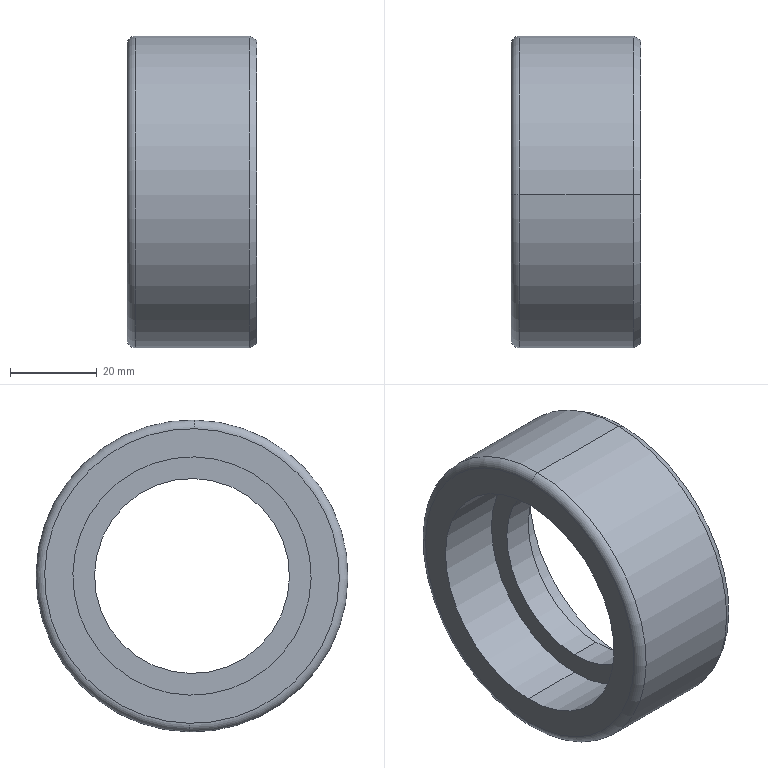Component | SolidWorks | 216InnerTubeAssembly-1_BearingPressSleeve1-1 | 1 solid | 16 faces | box 30 x 72 x 72 mm | volume 52368 mm3 | cylinder 8 | plane 4 | cone 2 | torus 2 | commonest cylinder face diameters 72 x2 60 x2 45 x2 55 x2 | material Alloy Steel
build123d program:
from build123d import *


with BuildPart() as part:
    # Model → Revolve1 (revolve)
    with BuildSketch(Plane.XY, mode=Mode.PRIVATE) as revolve1_sk:
        with BuildLine():
            Line((14.999, 22.5), (21.999, 22.5))
            Line((21.999, 22.5), (21.999, 27.5))
            Line((21.999, 27.5), (21.999, 30))
            Line((21.999, 30), (29.999, 30))
            Line((29.999, 30), (29.999, 35))
            Line((29.999, 35), (28.267, 36))
            Line((28.267, 36), (2, 36))
            ThreePointArc((2, 36), (0.5858, 35.414), (0, 34))
            Line((0, 34), (0, 27.5))
            Line((0, 27.5), (14.999, 27.5))
            Line((14.999, 27.5), (14.999, 22.5))
        make_face()
    revolve(revolve1_sk.sketch.rotate(Axis((0, 0, 0), (1, 0, 0)), 90), axis=Axis((0, 0, 0), (1, 0, 0)))


solid = part.part

# Placed as in the assembly
solid = solid.moved(Location((841.279, 0, 0), (0, 0, 0)))
STEP:
#1=COLOUR_RGB('',0.7922,0.8196,0.9333);
#2=FILL_AREA_STYLE_COLOUR('',#1);
#3=FILL_AREA_STYLE('',(#2));
#4=SURFACE_STYLE_FILL_AREA(#3);
#5=SURFACE_SIDE_STYLE('',(#4));
#6=SURFACE_STYLE_USAGE(.BOTH.,#5);
#7=PRESENTATION_STYLE_ASSIGNMENT((#6));
#8=CARTESIAN_POINT('',(34.234,-0.02545,1.417));
#9=VERTEX_POINT('',#8);
#10=CARTESIAN_POINT('',(34.234,0.02545,-1.417));
#11=VERTEX_POINT('',#10);
#12=CARTESIAN_POINT('',(34.234,-0.,0.));
#13=DIRECTION('',(-1.,-0.,0.));
#14=DIRECTION('',(0.,-0.01796,0.9998));
#15=AXIS2_PLACEMENT_3D('',#12,#13,#14);
#16=CIRCLE('',#15,1.417);
#17=EDGE_CURVE('',#9,#11,#16,.T.);
#18=ORIENTED_EDGE('',*,*,#17,.T.);
#19=CARTESIAN_POINT('',(33.2,0.02545,-1.417));
#20=VERTEX_POINT('',#19);
#21=CARTESIAN_POINT('',(33.121,0.02545,-1.417));
#22=DIRECTION('',(-1.,-0.,0.));
#23=VECTOR('',#22,39.37);
#24=LINE('',#21,#23);
#25=EDGE_CURVE('',#11,#20,#24,.T.);
#26=ORIENTED_EDGE('',*,*,#25,.T.);
#27=CARTESIAN_POINT('',(33.2,-0.02545,1.417));
#28=VERTEX_POINT('',#27);
#29=CARTESIAN_POINT('',(33.2,-0.,0.));
#30=DIRECTION('',(-1.,-0.,0.));
#31=DIRECTION('',(0.,-0.01796,0.9998));
#32=AXIS2_PLACEMENT_3D('',#29,#30,#31);
#33=CIRCLE('',#32,1.417);
#34=EDGE_CURVE('',#28,#20,#33,.T.);
#35=ORIENTED_EDGE('',*,*,#34,.F.);
#36=CARTESIAN_POINT('',(33.121,-0.02545,1.417));
#37=DIRECTION('',(-1.,-0.,0.));
#38=VECTOR('',#37,39.37);
#39=LINE('',#36,#38);
#40=EDGE_CURVE('',#9,#28,#39,.T.);
#41=ORIENTED_EDGE('',*,*,#40,.F.);
#42=EDGE_LOOP('',(#18,#26,#35,#41));
#43=FACE_OUTER_BOUND('',#42,.T.);
#44=CARTESIAN_POINT('',(33.121,-0.,0.));
#45=DIRECTION('',(-1.,-0.,0.));
#46=DIRECTION('',(0.,-0.01796,0.9998));
#47=AXIS2_PLACEMENT_3D('',#44,#45,#46);
#48=CYLINDRICAL_SURFACE('',#47,1.417);
#49=ADVANCED_FACE('',(#43),#48,.T.);
#50=CARTESIAN_POINT('',(34.302,-0.02474,1.378));
#51=VERTEX_POINT('',#50);
#52=CARTESIAN_POINT('',(34.302,0.02474,-1.378));
#53=VERTEX_POINT('',#52);
#54=CARTESIAN_POINT('',(34.302,-0.,0.));
#55=DIRECTION('',(-1.,-0.,0.));
#56=DIRECTION('',(0.,-0.01796,0.9998));
#57=AXIS2_PLACEMENT_3D('',#54,#55,#56);
#58=CIRCLE('',#57,1.378);
#59=EDGE_CURVE('',#51,#53,#58,.T.);
#60=ORIENTED_EDGE('',*,*,#59,.T.);
#61=CARTESIAN_POINT('',(34.302,0.02474,-1.378));
#62=DIRECTION('',(-0.866,0.008978,-0.4999));
#63=VECTOR('',#62,39.37);
#64=LINE('',#61,#63);
#65=EDGE_CURVE('',#53,#11,#64,.T.);
#66=ORIENTED_EDGE('',*,*,#65,.T.);
#67=ORIENTED_EDGE('',*,*,#17,.F.);
#68=CARTESIAN_POINT('',(34.302,-0.02474,1.378));
#69=DIRECTION('',(-0.866,-0.008978,0.4999));
#70=VECTOR('',#69,39.37);
#71=LINE('',#68,#70);
#72=EDGE_CURVE('',#51,#9,#71,.T.);
#73=ORIENTED_EDGE('',*,*,#72,.F.);
#74=EDGE_LOOP('',(#60,#66,#67,#73));
#75=FACE_OUTER_BOUND('',#74,.T.);
#76=CARTESIAN_POINT('',(34.302,-0.,0.));
#77=DIRECTION('',(-1.,-0.,0.));
#78=DIRECTION('',(0.,-0.01796,0.9998));
#79=AXIS2_PLACEMENT_3D('',#76,#77,#78);
#80=CONICAL_SURFACE('',#79,1.378,0.5236);
#81=ADVANCED_FACE('',(#75),#80,.T.);
#82=CARTESIAN_POINT('',(34.302,0.02121,-1.181));
#83=VERTEX_POINT('',#82);
#84=CARTESIAN_POINT('',(34.302,-0.02121,1.181));
#85=VERTEX_POINT('',#84);
#86=CARTESIAN_POINT('',(34.302,-0.,0.));
#87=DIRECTION('',(-1.,-0.,0.));
#88=DIRECTION('',(0.,-0.01796,0.9998));
#89=AXIS2_PLACEMENT_3D('',#86,#87,#88);
#90=CIRCLE('',#89,1.181);
#91=EDGE_CURVE('',#83,#85,#90,.T.);
#92=ORIENTED_EDGE('',*,*,#91,.F.);
#93=CARTESIAN_POINT('',(33.987,0.02121,-1.181));
#94=VERTEX_POINT('',#93);
#95=CARTESIAN_POINT('',(33.121,0.02121,-1.181));
#96=DIRECTION('',(-1.,-0.,0.));
#97=VECTOR('',#96,39.37);
#98=LINE('',#95,#97);
#99=EDGE_CURVE('',#83,#94,#98,.T.);
#100=ORIENTED_EDGE('',*,*,#99,.T.);
#101=CARTESIAN_POINT('',(33.987,-0.02121,1.181));
#102=VERTEX_POINT('',#101);
#103=CARTESIAN_POINT('',(33.987,-0.,0.));
#104=DIRECTION('',(-1.,-0.,0.));
#105=DIRECTION('',(0.,-0.01796,0.9998));
#106=AXIS2_PLACEMENT_3D('',#103,#104,#105);
#107=CIRCLE('',#106,1.181);
#108=EDGE_CURVE('',#94,#102,#107,.T.);
#109=ORIENTED_EDGE('',*,*,#108,.T.);
#110=CARTESIAN_POINT('',(33.121,-0.02121,1.181));
#111=DIRECTION('',(-1.,-0.,0.));
#112=VECTOR('',#111,39.37);
#113=LINE('',#110,#112);
#114=EDGE_CURVE('',#85,#102,#113,.T.);
#115=ORIENTED_EDGE('',*,*,#114,.F.);
#116=EDGE_LOOP('',(#92,#100,#109,#115));
#117=FACE_OUTER_BOUND('',#116,.T.);
#118=CARTESIAN_POINT('',(33.121,-0.,0.));
#119=DIRECTION('',(-1.,-0.,0.));
#120=DIRECTION('',(0.,-0.01796,0.9998));
#121=AXIS2_PLACEMENT_3D('',#118,#119,#120);
#122=CYLINDRICAL_SURFACE('',#121,1.181);
#123=ADVANCED_FACE('',(#117),#122,.F.);
#124=CARTESIAN_POINT('',(33.987,0.01591,-0.8857));
#125=VERTEX_POINT('',#124);
#126=CARTESIAN_POINT('',(33.987,-0.01591,0.8857));
#127=VERTEX_POINT('',#126);
#128=CARTESIAN_POINT('',(33.987,-0.,0.));
#129=DIRECTION('',(-1.,-0.,0.));
#130=DIRECTION('',(0.,-0.01796,0.9998));
#131=AXIS2_PLACEMENT_3D('',#128,#129,#130);
#132=CIRCLE('',#131,0.8858);
#133=EDGE_CURVE('',#125,#127,#132,.T.);
#134=ORIENTED_EDGE('',*,*,#133,.F.);
#135=CARTESIAN_POINT('',(33.712,0.01591,-0.8857));
#136=VERTEX_POINT('',#135);
#137=CARTESIAN_POINT('',(33.121,0.01591,-0.8857));
#138=DIRECTION('',(-1.,-0.,0.));
#139=VECTOR('',#138,39.37);
#140=LINE('',#137,#139);
#141=EDGE_CURVE('',#125,#136,#140,.T.);
#142=ORIENTED_EDGE('',*,*,#141,.T.);
#143=CARTESIAN_POINT('',(33.712,-0.01591,0.8857));
#144=VERTEX_POINT('',#143);
#145=CARTESIAN_POINT('',(33.712,-0.,0.));
#146=DIRECTION('',(-1.,-0.,0.));
#147=DIRECTION('',(0.,-0.01796,0.9998));
#148=AXIS2_PLACEMENT_3D('',#145,#146,#147);
#149=CIRCLE('',#148,0.8858);
#150=EDGE_CURVE('',#136,#144,#149,.T.);
#151=ORIENTED_EDGE('',*,*,#150,.T.);
#152=CARTESIAN_POINT('',(33.121,-0.01591,0.8857));
#153=DIRECTION('',(-1.,-0.,0.));
#154=VECTOR('',#153,39.37);
#155=LINE('',#152,#154);
#156=EDGE_CURVE('',#127,#144,#155,.T.);
#157=ORIENTED_EDGE('',*,*,#156,.F.);
#158=EDGE_LOOP('',(#134,#142,#151,#157));
#159=FACE_OUTER_BOUND('',#158,.T.);
#160=CARTESIAN_POINT('',(33.121,-0.,0.));
#161=DIRECTION('',(-1.,-0.,0.));
#162=DIRECTION('',(0.,-0.01796,0.9998));
#163=AXIS2_PLACEMENT_3D('',#160,#161,#162);
#164=CYLINDRICAL_SURFACE('',#163,0.8858);
#165=ADVANCED_FACE('',(#159),#164,.F.);
#166=CARTESIAN_POINT('',(33.712,0.01944,-1.083));
#167=VERTEX_POINT('',#166);
#168=CARTESIAN_POINT('',(33.712,-0.01944,1.083));
#169=VERTEX_POINT('',#168);
#170=CARTESIAN_POINT('',(33.712,-0.,0.));
#171=DIRECTION('',(-1.,-0.,0.));
#172=DIRECTION('',(0.,-0.01796,0.9998));
#173=AXIS2_PLACEMENT_3D('',#170,#171,#172);
#174=CIRCLE('',#173,1.083);
#175=EDGE_CURVE('',#167,#169,#174,.T.);
#176=ORIENTED_EDGE('',*,*,#175,.F.);
#177=CARTESIAN_POINT('',(33.121,0.01944,-1.083));
#178=VERTEX_POINT('',#177);
#179=CARTESIAN_POINT('',(33.121,0.01944,-1.083));
#180=DIRECTION('',(-1.,-0.,0.));
#181=VECTOR('',#180,39.37);
#182=LINE('',#179,#181);
#183=EDGE_CURVE('',#167,#178,#182,.T.);
#184=ORIENTED_EDGE('',*,*,#183,.T.);
#185=CARTESIAN_POINT('',(33.121,-0.01944,1.083));
#186=VERTEX_POINT('',#185);
#187=CARTESIAN_POINT('',(33.121,-0.,0.));
#188=DIRECTION('',(-1.,-0.,0.));
#189=DIRECTION('',(0.,-0.01796,0.9998));
#190=AXIS2_PLACEMENT_3D('',#187,#188,#189);
#191=CIRCLE('',#190,1.083);
#192=EDGE_CURVE('',#178,#186,#191,.T.);
#193=ORIENTED_EDGE('',*,*,#192,.T.);
#194=CARTESIAN_POINT('',(33.121,-0.01944,1.083));
#195=DIRECTION('',(-1.,-0.,0.));
#196=VECTOR('',#195,39.37);
#197=LINE('',#194,#196);
#198=EDGE_CURVE('',#169,#186,#197,.T.);
#199=ORIENTED_EDGE('',*,*,#198,.F.);
#200=EDGE_LOOP('',(#176,#184,#193,#199));
#201=FACE_OUTER_BOUND('',#200,.T.);
#202=CARTESIAN_POINT('',(33.121,-0.,0.));
#203=DIRECTION('',(-1.,-0.,0.));
#204=DIRECTION('',(0.,-0.01796,0.9998));
#205=AXIS2_PLACEMENT_3D('',#202,#203,#204);
#206=CYLINDRICAL_SURFACE('',#205,1.083);
#207=ADVANCED_FACE('',(#201),#206,.F.);
#208=ORIENTED_EDGE('',*,*,#34,.T.);
#209=CARTESIAN_POINT('',(33.121,0.02404,-1.338));
#210=VERTEX_POINT('',#209);
#211=CARTESIAN_POINT('',(33.2,0.02404,-1.338));
#212=DIRECTION('',(0.,0.9998,0.01796));
#213=DIRECTION('',(0.,-0.01796,0.9998));
#214=AXIS2_PLACEMENT_3D('',#211,#212,#213);
#215=CIRCLE('',#214,0.07874);
#216=EDGE_CURVE('',#20,#210,#215,.T.);
#217=ORIENTED_EDGE('',*,*,#216,.T.);
#218=CARTESIAN_POINT('',(33.121,-0.02404,1.338));
#219=VERTEX_POINT('',#218);
#220=CARTESIAN_POINT('',(33.121,-0.,0.));
#221=DIRECTION('',(-1.,-0.,0.));
#222=DIRECTION('',(0.,-0.01796,0.9998));
#223=AXIS2_PLACEMENT_3D('',#220,#221,#222);
#224=CIRCLE('',#223,1.339);
#225=EDGE_CURVE('',#219,#210,#224,.T.);
#226=ORIENTED_EDGE('',*,*,#225,.F.);
#227=CARTESIAN_POINT('',(33.2,-0.02404,1.338));
#228=DIRECTION('',(-0.,-0.9998,-0.01796));
#229=DIRECTION('',(0.,0.01796,-0.9998));
#230=AXIS2_PLACEMENT_3D('',#227,#228,#229);
#231=CIRCLE('',#230,0.07874);
#232=EDGE_CURVE('',#28,#219,#231,.T.);
#233=ORIENTED_EDGE('',*,*,#232,.F.);
#234=EDGE_LOOP('',(#208,#217,#226,#233));
#235=FACE_OUTER_BOUND('',#234,.T.);
#236=CARTESIAN_POINT('',(33.2,-0.,0.));
#237=DIRECTION('',(-1.,-0.,0.));
#238=DIRECTION('',(0.,-0.01796,0.9998));
#239=AXIS2_PLACEMENT_3D('',#236,#237,#238);
#240=TOROIDAL_SURFACE('',#239,1.339,0.07874);
#241=ADVANCED_FACE('',(#235),#240,.T.);
#242=ORIENTED_EDGE('',*,*,#216,.F.);
#243=CARTESIAN_POINT('',(33.2,-0.,0.));
#244=DIRECTION('',(-1.,-0.,0.));
#245=DIRECTION('',(0.,-0.01796,0.9998));
#246=AXIS2_PLACEMENT_3D('',#243,#244,#245);
#247=CIRCLE('',#246,1.417);
#248=EDGE_CURVE('',#20,#28,#247,.T.);
#249=ORIENTED_EDGE('',*,*,#248,.T.);
#250=ORIENTED_EDGE('',*,*,#232,.T.);
#251=CARTESIAN_POINT('',(33.121,-0.,0.));
#252=DIRECTION('',(-1.,-0.,0.));
#253=DIRECTION('',(0.,-0.01796,0.9998));
#254=AXIS2_PLACEMENT_3D('',#251,#252,#253);
#255=CIRCLE('',#254,1.339);
#256=EDGE_CURVE('',#210,#219,#255,.T.);
#257=ORIENTED_EDGE('',*,*,#256,.F.);
#258=EDGE_LOOP('',(#242,#249,#250,#257));
#259=FACE_OUTER_BOUND('',#258,.T.);
#260=CARTESIAN_POINT('',(33.2,-0.,0.));
#261=DIRECTION('',(-1.,-0.,0.));
#262=DIRECTION('',(0.,-0.01796,0.9998));
#263=AXIS2_PLACEMENT_3D('',#260,#261,#262);
#264=TOROIDAL_SURFACE('',#263,1.339,0.07874);
#265=ADVANCED_FACE('',(#259),#264,.T.);
#266=ORIENTED_EDGE('',*,*,#225,.T.);
#267=ORIENTED_EDGE('',*,*,#256,.T.);
#268=EDGE_LOOP('',(#266,#267));
#269=FACE_OUTER_BOUND('',#268,.T.);
#270=CARTESIAN_POINT('',(33.121,-0.,0.));
#271=DIRECTION('',(-1.,-0.,0.));
#272=DIRECTION('',(0.,-0.01796,0.9998));
#273=AXIS2_PLACEMENT_3D('',#270,#271,#272);
#274=CIRCLE('',#273,1.083);
#275=EDGE_CURVE('',#186,#178,#274,.T.);
#276=ORIENTED_EDGE('',*,*,#275,.F.);
#277=ORIENTED_EDGE('',*,*,#192,.F.);
#278=EDGE_LOOP('',(#276,#277));
#279=FACE_BOUND('',#278,.T.);
#280=CARTESIAN_POINT('',(33.121,-0.,0.));
#281=DIRECTION('',(-1.,-0.,0.));
#282=DIRECTION('',(0.,-0.01796,0.9998));
#283=AXIS2_PLACEMENT_3D('',#280,#281,#282);
#284=PLANE('',#283);
#285=ADVANCED_FACE('',(#269,#279),#284,.T.);
#286=ORIENTED_EDGE('',*,*,#183,.F.);
#287=CARTESIAN_POINT('',(33.712,-0.,0.));
#288=DIRECTION('',(-1.,-0.,0.));
#289=DIRECTION('',(0.,-0.01796,0.9998));
#290=AXIS2_PLACEMENT_3D('',#287,#288,#289);
#291=CIRCLE('',#290,1.083);
#292=EDGE_CURVE('',#169,#167,#291,.T.);
#293=ORIENTED_EDGE('',*,*,#292,.F.);
#294=ORIENTED_EDGE('',*,*,#198,.T.);
#295=ORIENTED_EDGE('',*,*,#275,.T.);
#296=EDGE_LOOP('',(#286,#293,#294,#295));
#297=FACE_OUTER_BOUND('',#296,.T.);
#298=CARTESIAN_POINT('',(33.121,-0.,0.));
#299=DIRECTION('',(-1.,-0.,0.));
#300=DIRECTION('',(0.,-0.01796,0.9998));
#301=AXIS2_PLACEMENT_3D('',#298,#299,#300);
#302=CYLINDRICAL_SURFACE('',#301,1.083);
#303=ADVANCED_FACE('',(#297),#302,.F.);
#304=ORIENTED_EDGE('',*,*,#292,.T.);
#305=ORIENTED_EDGE('',*,*,#175,.T.);
#306=EDGE_LOOP('',(#304,#305));
#307=FACE_OUTER_BOUND('',#306,.T.);
#308=CARTESIAN_POINT('',(33.712,-0.,0.));
#309=DIRECTION('',(-1.,-0.,0.));
#310=DIRECTION('',(0.,-0.01796,0.9998));
#311=AXIS2_PLACEMENT_3D('',#308,#309,#310);
#312=CIRCLE('',#311,0.8858);
#313=EDGE_CURVE('',#144,#136,#312,.T.);
#314=ORIENTED_EDGE('',*,*,#313,.F.);
#315=ORIENTED_EDGE('',*,*,#150,.F.);
#316=EDGE_LOOP('',(#314,#315));
#317=FACE_BOUND('',#316,.T.);
#318=CARTESIAN_POINT('',(33.712,-0.,0.));
#319=DIRECTION('',(-1.,-0.,0.));
#320=DIRECTION('',(0.,-0.01796,0.9998));
#321=AXIS2_PLACEMENT_3D('',#318,#319,#320);
#322=PLANE('',#321);
#323=ADVANCED_FACE('',(#307,#317),#322,.T.);
#324=ORIENTED_EDGE('',*,*,#141,.F.);
#325=CARTESIAN_POINT('',(33.987,-0.,0.));
#326=DIRECTION('',(-1.,-0.,0.));
#327=DIRECTION('',(0.,-0.01796,0.9998));
#328=AXIS2_PLACEMENT_3D('',#325,#326,#327);
#329=CIRCLE('',#328,0.8858);
#330=EDGE_CURVE('',#127,#125,#329,.T.);
#331=ORIENTED_EDGE('',*,*,#330,.F.);
#332=ORIENTED_EDGE('',*,*,#156,.T.);
#333=ORIENTED_EDGE('',*,*,#313,.T.);
#334=EDGE_LOOP('',(#324,#331,#332,#333));
#335=FACE_OUTER_BOUND('',#334,.T.);
#336=CARTESIAN_POINT('',(33.121,-0.,0.));
#337=DIRECTION('',(-1.,-0.,0.));
#338=DIRECTION('',(0.,-0.01796,0.9998));
#339=AXIS2_PLACEMENT_3D('',#336,#337,#338);
#340=CYLINDRICAL_SURFACE('',#339,0.8858);
#341=ADVANCED_FACE('',(#335),#340,.F.);
#342=CARTESIAN_POINT('',(33.987,-0.,0.));
#343=DIRECTION('',(-1.,-0.,0.));
#344=DIRECTION('',(0.,-0.01796,0.9998));
#345=AXIS2_PLACEMENT_3D('',#342,#343,#344);
#346=CIRCLE('',#345,1.181);
#347=EDGE_CURVE('',#102,#94,#346,.T.);
#348=ORIENTED_EDGE('',*,*,#347,.F.);
#349=ORIENTED_EDGE('',*,*,#108,.F.);
#350=EDGE_LOOP('',(#348,#349));
#351=FACE_OUTER_BOUND('',#350,.T.);
#352=ORIENTED_EDGE('',*,*,#330,.T.);
#353=ORIENTED_EDGE('',*,*,#133,.T.);
#354=EDGE_LOOP('',(#352,#353));
#355=FACE_BOUND('',#354,.T.);
#356=CARTESIAN_POINT('',(33.987,-0.,0.));
#357=DIRECTION('',(-1.,-0.,0.));
#358=DIRECTION('',(0.,-0.01796,0.9998));
#359=AXIS2_PLACEMENT_3D('',#356,#357,#358);
#360=PLANE('',#359);
#361=ADVANCED_FACE('',(#351,#355),#360,.F.);
#362=ORIENTED_EDGE('',*,*,#99,.F.);
#363=CARTESIAN_POINT('',(34.302,-0.,0.));
#364=DIRECTION('',(-1.,-0.,0.));
#365=DIRECTION('',(0.,-0.01796,0.9998));
#366=AXIS2_PLACEMENT_3D('',#363,#364,#365);
#367=CIRCLE('',#366,1.181);
#368=EDGE_CURVE('',#85,#83,#367,.T.);
#369=ORIENTED_EDGE('',*,*,#368,.F.);
#370=ORIENTED_EDGE('',*,*,#114,.T.);
#371=ORIENTED_EDGE('',*,*,#347,.T.);
#372=EDGE_LOOP('',(#362,#369,#370,#371));
#373=FACE_OUTER_BOUND('',#372,.T.);
#374=CARTESIAN_POINT('',(33.121,-0.,0.));
#375=DIRECTION('',(-1.,-0.,0.));
#376=DIRECTION('',(0.,-0.01796,0.9998));
#377=AXIS2_PLACEMENT_3D('',#374,#375,#376);
#378=CYLINDRICAL_SURFACE('',#377,1.181);
#379=ADVANCED_FACE('',(#373),#378,.F.);
#380=ORIENTED_EDGE('',*,*,#59,.F.);
#381=CARTESIAN_POINT('',(34.302,-0.,0.));
#382=DIRECTION('',(-1.,-0.,0.));
#383=DIRECTION('',(0.,-0.01796,0.9998));
#384=AXIS2_PLACEMENT_3D('',#381,#382,#383);
#385=CIRCLE('',#384,1.378);
#386=EDGE_CURVE('',#53,#51,#385,.T.);
#387=ORIENTED_EDGE('',*,*,#386,.F.);
#388=EDGE_LOOP('',(#380,#387));
#389=FACE_OUTER_BOUND('',#388,.T.);
#390=ORIENTED_EDGE('',*,*,#368,.T.);
#391=ORIENTED_EDGE('',*,*,#91,.T.);
#392=EDGE_LOOP('',(#390,#391));
#393=FACE_BOUND('',#392,.T.);
#394=CARTESIAN_POINT('',(34.302,-0.,0.));
#395=DIRECTION('',(-1.,-0.,0.));
#396=DIRECTION('',(0.,-0.01796,0.9998));
#397=AXIS2_PLACEMENT_3D('',#394,#395,#396);
#398=PLANE('',#397);
#399=ADVANCED_FACE('',(#389,#393),#398,.F.);
#400=ORIENTED_EDGE('',*,*,#65,.F.);
#401=ORIENTED_EDGE('',*,*,#386,.T.);
#402=ORIENTED_EDGE('',*,*,#72,.T.);
#403=CARTESIAN_POINT('',(34.234,-0.,0.));
#404=DIRECTION('',(-1.,-0.,0.));
#405=DIRECTION('',(0.,-0.01796,0.9998));
#406=AXIS2_PLACEMENT_3D('',#403,#404,#405);
#407=CIRCLE('',#406,1.417);
#408=EDGE_CURVE('',#11,#9,#407,.T.);
#409=ORIENTED_EDGE('',*,*,#408,.F.);
#410=EDGE_LOOP('',(#400,#401,#402,#409));
#411=FACE_OUTER_BOUND('',#410,.T.);
#412=CARTESIAN_POINT('',(34.302,-0.,0.));
#413=DIRECTION('',(-1.,-0.,0.));
#414=DIRECTION('',(0.,-0.01796,0.9998));
#415=AXIS2_PLACEMENT_3D('',#412,#413,#414);
#416=CONICAL_SURFACE('',#415,1.378,0.5236);
#417=ADVANCED_FACE('',(#411),#416,.T.);
#418=ORIENTED_EDGE('',*,*,#25,.F.);
#419=ORIENTED_EDGE('',*,*,#408,.T.);
#420=ORIENTED_EDGE('',*,*,#40,.T.);
#421=ORIENTED_EDGE('',*,*,#248,.F.);
#422=EDGE_LOOP('',(#418,#419,#420,#421));
#423=FACE_OUTER_BOUND('',#422,.T.);
#424=CARTESIAN_POINT('',(33.121,-0.,0.));
#425=DIRECTION('',(-1.,-0.,0.));
#426=DIRECTION('',(0.,-0.01796,0.9998));
#427=AXIS2_PLACEMENT_3D('',#424,#425,#426);
#428=CYLINDRICAL_SURFACE('',#427,1.417);
#429=ADVANCED_FACE('',(#423),#428,.T.);
#430=CLOSED_SHELL('',(#49,#81,#123,#165,#207,#241,#265,#285,#303,#323,#341,#361,#379,#399,#417,#429));
#431=MANIFOLD_SOLID_BREP('',#430);
#432=STYLED_ITEM('',(#7),#431);
#433=PRESENTATION_LAYER_ASSIGNMENT('','',(#432));
#434=(LENGTH_UNIT()NAMED_UNIT(*)SI_UNIT($,.METRE.));
#435=LENGTH_MEASURE_WITH_UNIT(LENGTH_MEASURE(0.0254),#434);
#436=DIMENSIONAL_EXPONENTS(1.,0.,0.,0.,0.,0.,0.);
#437=(CONVERSION_BASED_UNIT('',#435)LENGTH_UNIT()NAMED_UNIT(#436));
#438=UNCERTAINTY_MEASURE_WITH_UNIT(LENGTH_MEASURE(0.00001),#437,'','');
#439=(NAMED_UNIT(*)PLANE_ANGLE_UNIT()SI_UNIT($,.RADIAN.));
#440=(NAMED_UNIT(*)SI_UNIT($,.STERADIAN.)SOLID_ANGLE_UNIT());
#441=(GEOMETRIC_REPRESENTATION_CONTEXT(3)GLOBAL_UNCERTAINTY_ASSIGNED_CONTEXT((#438))GLOBAL_UNIT_ASSIGNED_CONTEXT((#437,#439,#440))REPRESENTATION_CONTEXT('',''));
#442=MECHANICAL_DESIGN_GEOMETRIC_PRESENTATION_REPRESENTATION('',(#432),#441);
#443=CARTESIAN_POINT('',(0.,0.,0.));
#444=DIRECTION('',(0.,0.,1.));
#445=DIRECTION('',(1.,0.,0.));
#446=AXIS2_PLACEMENT_3D('',#443,#444,#445);
#447=(LENGTH_UNIT()NAMED_UNIT(*)SI_UNIT($,.METRE.));
#448=LENGTH_MEASURE_WITH_UNIT(LENGTH_MEASURE(0.0254),#447);
#449=DIMENSIONAL_EXPONENTS(1.,0.,0.,0.,0.,0.,0.);
#450=(CONVERSION_BASED_UNIT('',#448)LENGTH_UNIT()NAMED_UNIT(#449));
#451=UNCERTAINTY_MEASURE_WITH_UNIT(LENGTH_MEASURE(0.00001),#450,'','');
#452=(NAMED_UNIT(*)PLANE_ANGLE_UNIT()SI_UNIT($,.RADIAN.));
#453=(NAMED_UNIT(*)SI_UNIT($,.STERADIAN.)SOLID_ANGLE_UNIT());
#454=(GEOMETRIC_REPRESENTATION_CONTEXT(3)GLOBAL_UNCERTAINTY_ASSIGNED_CONTEXT((#451))GLOBAL_UNIT_ASSIGNED_CONTEXT((#450,#452,#453))REPRESENTATION_CONTEXT('',''));
#455=ADVANCED_BREP_SHAPE_REPRESENTATION('',(#431,#446),#454);